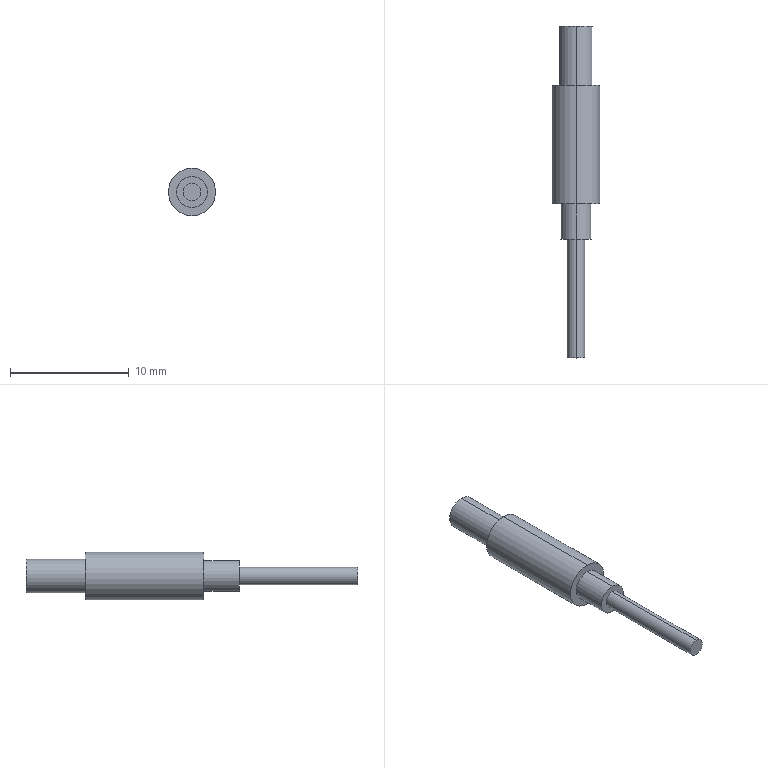Component | SolidWorks | FiberOpticHeadM4x10-1 | 1 solid | 13 faces | box 4 x 28 x 4 mm | volume 189 mm3 | cylinder 8 | plane 5 | commonest cylinder face diameters 2.8 x2 4 x2 2.6 x2 1.47 x2
build123d program:
from build123d import *


with BuildPart() as part:
    # Sketch1 → Revolve1 (revolve)
    with BuildSketch(Plane.XY, mode=Mode.PRIVATE) as revolve1_sk:
        Polygon((0, 0), (0.735, 0), (0.735, 10), (1.3, 10), (1.3, 13), (2, 13), (2, 23), (1.4, 23), (1.4, 28), (0, 28), align=None)
    revolve(revolve1_sk.sketch.rotate(Axis((0, 0, 0), (0, -1, 0)), 90), axis=Axis((0, 0, 0), (0, -1, 0)))


solid = part.part

# Placed as in the assembly
solid = solid.moved(Location((20.665, -23.632, -215.315), (0, 0, 0)))
STEP:
#1=COLOUR_RGB('',0.7922,0.8196,0.9333);
#2=FILL_AREA_STYLE_COLOUR('',#1);
#3=FILL_AREA_STYLE('',(#2));
#4=SURFACE_STYLE_FILL_AREA(#3);
#5=SURFACE_SIDE_STYLE('',(#4));
#6=SURFACE_STYLE_USAGE(.BOTH.,#5);
#7=PRESENTATION_STYLE_ASSIGNMENT((#6));
#8=CARTESIAN_POINT('',(0.8136,-0.02487,-8.422));
#9=VERTEX_POINT('',#8);
#10=CARTESIAN_POINT('',(0.8136,-0.02487,-8.532));
#11=VERTEX_POINT('',#10);
#12=CARTESIAN_POINT('',(0.8136,-0.02487,-8.477));
#13=DIRECTION('',(0.,1.,0.));
#14=DIRECTION('',(0.,0.,1.));
#15=AXIS2_PLACEMENT_3D('',#12,#13,#14);
#16=CIRCLE('',#15,0.05512);
#17=EDGE_CURVE('',#9,#11,#16,.T.);
#18=ORIENTED_EDGE('',*,*,#17,.T.);
#19=CARTESIAN_POINT('',(0.8136,0.172,-8.532));
#20=VERTEX_POINT('',#19);
#21=CARTESIAN_POINT('',(0.8136,-0.9304,-8.532));
#22=DIRECTION('',(0.,1.,0.));
#23=VECTOR('',#22,39.37);
#24=LINE('',#21,#23);
#25=EDGE_CURVE('',#11,#20,#24,.T.);
#26=ORIENTED_EDGE('',*,*,#25,.T.);
#27=CARTESIAN_POINT('',(0.8136,0.172,-8.422));
#28=VERTEX_POINT('',#27);
#29=CARTESIAN_POINT('',(0.8136,0.172,-8.477));
#30=DIRECTION('',(0.,1.,0.));
#31=DIRECTION('',(0.,0.,1.));
#32=AXIS2_PLACEMENT_3D('',#29,#30,#31);
#33=CIRCLE('',#32,0.05512);
#34=EDGE_CURVE('',#28,#20,#33,.T.);
#35=ORIENTED_EDGE('',*,*,#34,.F.);
#36=CARTESIAN_POINT('',(0.8136,-0.9304,-8.422));
#37=DIRECTION('',(0.,1.,0.));
#38=VECTOR('',#37,39.37);
#39=LINE('',#36,#38);
#40=EDGE_CURVE('',#9,#28,#39,.T.);
#41=ORIENTED_EDGE('',*,*,#40,.F.);
#42=EDGE_LOOP('',(#18,#26,#35,#41));
#43=FACE_OUTER_BOUND('',#42,.T.);
#44=CARTESIAN_POINT('',(0.8136,-0.9304,-8.477));
#45=DIRECTION('',(0.,1.,0.));
#46=DIRECTION('',(0.,0.,1.));
#47=AXIS2_PLACEMENT_3D('',#44,#45,#46);
#48=CYLINDRICAL_SURFACE('',#47,0.05512);
#49=ADVANCED_FACE('',(#43),#48,.T.);
#50=CARTESIAN_POINT('',(0.8136,-0.4186,-8.398));
#51=VERTEX_POINT('',#50);
#52=CARTESIAN_POINT('',(0.8136,-0.4186,-8.556));
#53=VERTEX_POINT('',#52);
#54=CARTESIAN_POINT('',(0.8136,-0.4186,-8.477));
#55=DIRECTION('',(0.,1.,0.));
#56=DIRECTION('',(0.,0.,1.));
#57=AXIS2_PLACEMENT_3D('',#54,#55,#56);
#58=CIRCLE('',#57,0.07874);
#59=EDGE_CURVE('',#51,#53,#58,.T.);
#60=ORIENTED_EDGE('',*,*,#59,.T.);
#61=CARTESIAN_POINT('',(0.8136,-0.02487,-8.556));
#62=VERTEX_POINT('',#61);
#63=CARTESIAN_POINT('',(0.8136,-0.9304,-8.556));
#64=DIRECTION('',(0.,1.,0.));
#65=VECTOR('',#64,39.37);
#66=LINE('',#63,#65);
#67=EDGE_CURVE('',#53,#62,#66,.T.);
#68=ORIENTED_EDGE('',*,*,#67,.T.);
#69=CARTESIAN_POINT('',(0.8136,-0.02487,-8.398));
#70=VERTEX_POINT('',#69);
#71=CARTESIAN_POINT('',(0.8136,-0.02487,-8.477));
#72=DIRECTION('',(0.,1.,0.));
#73=DIRECTION('',(0.,0.,1.));
#74=AXIS2_PLACEMENT_3D('',#71,#72,#73);
#75=CIRCLE('',#74,0.07874);
#76=EDGE_CURVE('',#70,#62,#75,.T.);
#77=ORIENTED_EDGE('',*,*,#76,.F.);
#78=CARTESIAN_POINT('',(0.8136,-0.9304,-8.398));
#79=DIRECTION('',(0.,1.,0.));
#80=VECTOR('',#79,39.37);
#81=LINE('',#78,#80);
#82=EDGE_CURVE('',#51,#70,#81,.T.);
#83=ORIENTED_EDGE('',*,*,#82,.F.);
#84=EDGE_LOOP('',(#60,#68,#77,#83));
#85=FACE_OUTER_BOUND('',#84,.T.);
#86=CARTESIAN_POINT('',(0.8136,-0.9304,-8.477));
#87=DIRECTION('',(0.,1.,0.));
#88=DIRECTION('',(0.,0.,1.));
#89=AXIS2_PLACEMENT_3D('',#86,#87,#88);
#90=CYLINDRICAL_SURFACE('',#89,0.07874);
#91=ADVANCED_FACE('',(#85),#90,.T.);
#92=CARTESIAN_POINT('',(0.8136,-0.5367,-8.426));
#93=VERTEX_POINT('',#92);
#94=CARTESIAN_POINT('',(0.8136,-0.5367,-8.528));
#95=VERTEX_POINT('',#94);
#96=CARTESIAN_POINT('',(0.8136,-0.5367,-8.477));
#97=DIRECTION('',(0.,1.,0.));
#98=DIRECTION('',(0.,0.,1.));
#99=AXIS2_PLACEMENT_3D('',#96,#97,#98);
#100=CIRCLE('',#99,0.05118);
#101=EDGE_CURVE('',#93,#95,#100,.T.);
#102=ORIENTED_EDGE('',*,*,#101,.T.);
#103=CARTESIAN_POINT('',(0.8136,-0.4186,-8.528));
#104=VERTEX_POINT('',#103);
#105=CARTESIAN_POINT('',(0.8136,-0.9304,-8.528));
#106=DIRECTION('',(0.,1.,0.));
#107=VECTOR('',#106,39.37);
#108=LINE('',#105,#107);
#109=EDGE_CURVE('',#95,#104,#108,.T.);
#110=ORIENTED_EDGE('',*,*,#109,.T.);
#111=CARTESIAN_POINT('',(0.8136,-0.4186,-8.426));
#112=VERTEX_POINT('',#111);
#113=CARTESIAN_POINT('',(0.8136,-0.4186,-8.477));
#114=DIRECTION('',(0.,1.,0.));
#115=DIRECTION('',(0.,0.,1.));
#116=AXIS2_PLACEMENT_3D('',#113,#114,#115);
#117=CIRCLE('',#116,0.05118);
#118=EDGE_CURVE('',#112,#104,#117,.T.);
#119=ORIENTED_EDGE('',*,*,#118,.F.);
#120=CARTESIAN_POINT('',(0.8136,-0.9304,-8.426));
#121=DIRECTION('',(0.,1.,0.));
#122=VECTOR('',#121,39.37);
#123=LINE('',#120,#122);
#124=EDGE_CURVE('',#93,#112,#123,.T.);
#125=ORIENTED_EDGE('',*,*,#124,.F.);
#126=EDGE_LOOP('',(#102,#110,#119,#125));
#127=FACE_OUTER_BOUND('',#126,.T.);
#128=CARTESIAN_POINT('',(0.8136,-0.9304,-8.477));
#129=DIRECTION('',(0.,1.,0.));
#130=DIRECTION('',(0.,0.,1.));
#131=AXIS2_PLACEMENT_3D('',#128,#129,#130);
#132=CYLINDRICAL_SURFACE('',#131,0.05118);
#133=ADVANCED_FACE('',(#127),#132,.T.);
#134=CARTESIAN_POINT('',(0.8136,-0.9304,-8.448));
#135=VERTEX_POINT('',#134);
#136=CARTESIAN_POINT('',(0.8136,-0.9304,-8.506));
#137=VERTEX_POINT('',#136);
#138=CARTESIAN_POINT('',(0.8136,-0.9304,-8.477));
#139=DIRECTION('',(0.,1.,0.));
#140=DIRECTION('',(0.,0.,1.));
#141=AXIS2_PLACEMENT_3D('',#138,#139,#140);
#142=CIRCLE('',#141,0.02894);
#143=EDGE_CURVE('',#135,#137,#142,.T.);
#144=ORIENTED_EDGE('',*,*,#143,.T.);
#145=CARTESIAN_POINT('',(0.8136,-0.5367,-8.506));
#146=VERTEX_POINT('',#145);
#147=CARTESIAN_POINT('',(0.8136,-0.9304,-8.506));
#148=DIRECTION('',(0.,1.,0.));
#149=VECTOR('',#148,39.37);
#150=LINE('',#147,#149);
#151=EDGE_CURVE('',#137,#146,#150,.T.);
#152=ORIENTED_EDGE('',*,*,#151,.T.);
#153=CARTESIAN_POINT('',(0.8136,-0.5367,-8.448));
#154=VERTEX_POINT('',#153);
#155=CARTESIAN_POINT('',(0.8136,-0.5367,-8.477));
#156=DIRECTION('',(0.,1.,0.));
#157=DIRECTION('',(0.,0.,1.));
#158=AXIS2_PLACEMENT_3D('',#155,#156,#157);
#159=CIRCLE('',#158,0.02894);
#160=EDGE_CURVE('',#154,#146,#159,.T.);
#161=ORIENTED_EDGE('',*,*,#160,.F.);
#162=CARTESIAN_POINT('',(0.8136,-0.9304,-8.448));
#163=DIRECTION('',(0.,1.,0.));
#164=VECTOR('',#163,39.37);
#165=LINE('',#162,#164);
#166=EDGE_CURVE('',#135,#154,#165,.T.);
#167=ORIENTED_EDGE('',*,*,#166,.F.);
#168=EDGE_LOOP('',(#144,#152,#161,#167));
#169=FACE_OUTER_BOUND('',#168,.T.);
#170=CARTESIAN_POINT('',(0.8136,-0.9304,-8.477));
#171=DIRECTION('',(0.,1.,0.));
#172=DIRECTION('',(0.,0.,1.));
#173=AXIS2_PLACEMENT_3D('',#170,#171,#172);
#174=CYLINDRICAL_SURFACE('',#173,0.02894);
#175=ADVANCED_FACE('',(#169),#174,.T.);
#176=ORIENTED_EDGE('',*,*,#143,.F.);
#177=CARTESIAN_POINT('',(0.8136,-0.9304,-8.477));
#178=DIRECTION('',(0.,1.,0.));
#179=DIRECTION('',(0.,0.,1.));
#180=AXIS2_PLACEMENT_3D('',#177,#178,#179);
#181=CIRCLE('',#180,0.02894);
#182=EDGE_CURVE('',#137,#135,#181,.T.);
#183=ORIENTED_EDGE('',*,*,#182,.F.);
#184=EDGE_LOOP('',(#176,#183));
#185=FACE_OUTER_BOUND('',#184,.T.);
#186=CARTESIAN_POINT('',(0.8136,-0.9304,-8.477));
#187=DIRECTION('',(0.,1.,0.));
#188=DIRECTION('',(0.,0.,1.));
#189=AXIS2_PLACEMENT_3D('',#186,#187,#188);
#190=PLANE('',#189);
#191=ADVANCED_FACE('',(#185),#190,.F.);
#192=ORIENTED_EDGE('',*,*,#151,.F.);
#193=ORIENTED_EDGE('',*,*,#182,.T.);
#194=ORIENTED_EDGE('',*,*,#166,.T.);
#195=CARTESIAN_POINT('',(0.8136,-0.5367,-8.477));
#196=DIRECTION('',(0.,1.,0.));
#197=DIRECTION('',(0.,0.,1.));
#198=AXIS2_PLACEMENT_3D('',#195,#196,#197);
#199=CIRCLE('',#198,0.02894);
#200=EDGE_CURVE('',#146,#154,#199,.T.);
#201=ORIENTED_EDGE('',*,*,#200,.F.);
#202=EDGE_LOOP('',(#192,#193,#194,#201));
#203=FACE_OUTER_BOUND('',#202,.T.);
#204=CARTESIAN_POINT('',(0.8136,-0.9304,-8.477));
#205=DIRECTION('',(0.,1.,0.));
#206=DIRECTION('',(0.,0.,1.));
#207=AXIS2_PLACEMENT_3D('',#204,#205,#206);
#208=CYLINDRICAL_SURFACE('',#207,0.02894);
#209=ADVANCED_FACE('',(#203),#208,.T.);
#210=ORIENTED_EDGE('',*,*,#101,.F.);
#211=CARTESIAN_POINT('',(0.8136,-0.5367,-8.477));
#212=DIRECTION('',(0.,1.,0.));
#213=DIRECTION('',(0.,0.,1.));
#214=AXIS2_PLACEMENT_3D('',#211,#212,#213);
#215=CIRCLE('',#214,0.05118);
#216=EDGE_CURVE('',#95,#93,#215,.T.);
#217=ORIENTED_EDGE('',*,*,#216,.F.);
#218=EDGE_LOOP('',(#210,#217));
#219=FACE_OUTER_BOUND('',#218,.T.);
#220=ORIENTED_EDGE('',*,*,#160,.T.);
#221=ORIENTED_EDGE('',*,*,#200,.T.);
#222=EDGE_LOOP('',(#220,#221));
#223=FACE_BOUND('',#222,.T.);
#224=CARTESIAN_POINT('',(0.8425,-0.5367,-8.477));
#225=DIRECTION('',(0.,1.,0.));
#226=DIRECTION('',(0.,0.,1.));
#227=AXIS2_PLACEMENT_3D('',#224,#225,#226);
#228=PLANE('',#227);
#229=ADVANCED_FACE('',(#219,#223),#228,.F.);
#230=ORIENTED_EDGE('',*,*,#109,.F.);
#231=ORIENTED_EDGE('',*,*,#216,.T.);
#232=ORIENTED_EDGE('',*,*,#124,.T.);
#233=CARTESIAN_POINT('',(0.8136,-0.4186,-8.477));
#234=DIRECTION('',(0.,1.,0.));
#235=DIRECTION('',(0.,0.,1.));
#236=AXIS2_PLACEMENT_3D('',#233,#234,#235);
#237=CIRCLE('',#236,0.05118);
#238=EDGE_CURVE('',#104,#112,#237,.T.);
#239=ORIENTED_EDGE('',*,*,#238,.F.);
#240=EDGE_LOOP('',(#230,#231,#232,#239));
#241=FACE_OUTER_BOUND('',#240,.T.);
#242=CARTESIAN_POINT('',(0.8136,-0.9304,-8.477));
#243=DIRECTION('',(0.,1.,0.));
#244=DIRECTION('',(0.,0.,1.));
#245=AXIS2_PLACEMENT_3D('',#242,#243,#244);
#246=CYLINDRICAL_SURFACE('',#245,0.05118);
#247=ADVANCED_FACE('',(#241),#246,.T.);
#248=ORIENTED_EDGE('',*,*,#59,.F.);
#249=CARTESIAN_POINT('',(0.8136,-0.4186,-8.477));
#250=DIRECTION('',(0.,1.,0.));
#251=DIRECTION('',(0.,0.,1.));
#252=AXIS2_PLACEMENT_3D('',#249,#250,#251);
#253=CIRCLE('',#252,0.07874);
#254=EDGE_CURVE('',#53,#51,#253,.T.);
#255=ORIENTED_EDGE('',*,*,#254,.F.);
#256=EDGE_LOOP('',(#248,#255));
#257=FACE_OUTER_BOUND('',#256,.T.);
#258=ORIENTED_EDGE('',*,*,#118,.T.);
#259=ORIENTED_EDGE('',*,*,#238,.T.);
#260=EDGE_LOOP('',(#258,#259));
#261=FACE_BOUND('',#260,.T.);
#262=CARTESIAN_POINT('',(0.8648,-0.4186,-8.477));
#263=DIRECTION('',(0.,1.,0.));
#264=DIRECTION('',(0.,0.,1.));
#265=AXIS2_PLACEMENT_3D('',#262,#263,#264);
#266=PLANE('',#265);
#267=ADVANCED_FACE('',(#257,#261),#266,.F.);
#268=ORIENTED_EDGE('',*,*,#67,.F.);
#269=ORIENTED_EDGE('',*,*,#254,.T.);
#270=ORIENTED_EDGE('',*,*,#82,.T.);
#271=CARTESIAN_POINT('',(0.8136,-0.02487,-8.477));
#272=DIRECTION('',(0.,1.,0.));
#273=DIRECTION('',(0.,0.,1.));
#274=AXIS2_PLACEMENT_3D('',#271,#272,#273);
#275=CIRCLE('',#274,0.07874);
#276=EDGE_CURVE('',#62,#70,#275,.T.);
#277=ORIENTED_EDGE('',*,*,#276,.F.);
#278=EDGE_LOOP('',(#268,#269,#270,#277));
#279=FACE_OUTER_BOUND('',#278,.T.);
#280=CARTESIAN_POINT('',(0.8136,-0.9304,-8.477));
#281=DIRECTION('',(0.,1.,0.));
#282=DIRECTION('',(0.,0.,1.));
#283=AXIS2_PLACEMENT_3D('',#280,#281,#282);
#284=CYLINDRICAL_SURFACE('',#283,0.07874);
#285=ADVANCED_FACE('',(#279),#284,.T.);
#286=ORIENTED_EDGE('',*,*,#17,.F.);
#287=CARTESIAN_POINT('',(0.8136,-0.02487,-8.477));
#288=DIRECTION('',(0.,1.,0.));
#289=DIRECTION('',(0.,0.,1.));
#290=AXIS2_PLACEMENT_3D('',#287,#288,#289);
#291=CIRCLE('',#290,0.05512);
#292=EDGE_CURVE('',#11,#9,#291,.T.);
#293=ORIENTED_EDGE('',*,*,#292,.F.);
#294=EDGE_LOOP('',(#286,#293));
#295=FACE_BOUND('',#294,.T.);
#296=ORIENTED_EDGE('',*,*,#76,.T.);
#297=ORIENTED_EDGE('',*,*,#276,.T.);
#298=EDGE_LOOP('',(#296,#297));
#299=FACE_OUTER_BOUND('',#298,.T.);
#300=CARTESIAN_POINT('',(0.8923,-0.02487,-8.477));
#301=DIRECTION('',(0.,-1.,0.));
#302=DIRECTION('',(0.,0.,-1.));
#303=AXIS2_PLACEMENT_3D('',#300,#301,#302);
#304=PLANE('',#303);
#305=ADVANCED_FACE('',(#295,#299),#304,.F.);
#306=ORIENTED_EDGE('',*,*,#25,.F.);
#307=ORIENTED_EDGE('',*,*,#292,.T.);
#308=ORIENTED_EDGE('',*,*,#40,.T.);
#309=CARTESIAN_POINT('',(0.8136,0.172,-8.477));
#310=DIRECTION('',(0.,1.,0.));
#311=DIRECTION('',(0.,0.,1.));
#312=AXIS2_PLACEMENT_3D('',#309,#310,#311);
#313=CIRCLE('',#312,0.05512);
#314=EDGE_CURVE('',#20,#28,#313,.T.);
#315=ORIENTED_EDGE('',*,*,#314,.F.);
#316=EDGE_LOOP('',(#306,#307,#308,#315));
#317=FACE_OUTER_BOUND('',#316,.T.);
#318=CARTESIAN_POINT('',(0.8136,-0.9304,-8.477));
#319=DIRECTION('',(0.,1.,0.));
#320=DIRECTION('',(0.,0.,1.));
#321=AXIS2_PLACEMENT_3D('',#318,#319,#320);
#322=CYLINDRICAL_SURFACE('',#321,0.05512);
#323=ADVANCED_FACE('',(#317),#322,.T.);
#324=ORIENTED_EDGE('',*,*,#34,.T.);
#325=ORIENTED_EDGE('',*,*,#314,.T.);
#326=EDGE_LOOP('',(#324,#325));
#327=FACE_OUTER_BOUND('',#326,.T.);
#328=CARTESIAN_POINT('',(0.8687,0.172,-8.477));
#329=DIRECTION('',(0.,-1.,0.));
#330=DIRECTION('',(0.,0.,-1.));
#331=AXIS2_PLACEMENT_3D('',#328,#329,#330);
#332=PLANE('',#331);
#333=ADVANCED_FACE('',(#327),#332,.F.);
#334=CLOSED_SHELL('',(#49,#91,#133,#175,#191,#209,#229,#247,#267,#285,#305,#323,#333));
#335=MANIFOLD_SOLID_BREP('',#334);
#336=STYLED_ITEM('',(#7),#335);
#337=(LENGTH_UNIT()NAMED_UNIT(*)SI_UNIT($,.METRE.));
#338=LENGTH_MEASURE_WITH_UNIT(LENGTH_MEASURE(0.0254),#337);
#339=DIMENSIONAL_EXPONENTS(1.,0.,0.,0.,0.,0.,0.);
#340=(CONVERSION_BASED_UNIT('',#338)LENGTH_UNIT()NAMED_UNIT(#339));
#341=UNCERTAINTY_MEASURE_WITH_UNIT(LENGTH_MEASURE(0.00001),#340,'','');
#342=(NAMED_UNIT(*)PLANE_ANGLE_UNIT()SI_UNIT($,.RADIAN.));
#343=(NAMED_UNIT(*)SI_UNIT($,.STERADIAN.)SOLID_ANGLE_UNIT());
#344=(GEOMETRIC_REPRESENTATION_CONTEXT(3)GLOBAL_UNCERTAINTY_ASSIGNED_CONTEXT((#341))GLOBAL_UNIT_ASSIGNED_CONTEXT((#340,#342,#343))REPRESENTATION_CONTEXT('',''));
#345=MECHANICAL_DESIGN_GEOMETRIC_PRESENTATION_REPRESENTATION('',(#336),#344);
#346=CARTESIAN_POINT('',(0.,0.,0.));
#347=DIRECTION('',(0.,0.,1.));
#348=DIRECTION('',(1.,0.,0.));
#349=AXIS2_PLACEMENT_3D('',#346,#347,#348);
#350=(LENGTH_UNIT()NAMED_UNIT(*)SI_UNIT($,.METRE.));
#351=LENGTH_MEASURE_WITH_UNIT(LENGTH_MEASURE(0.0254),#350);
#352=DIMENSIONAL_EXPONENTS(1.,0.,0.,0.,0.,0.,0.);
#353=(CONVERSION_BASED_UNIT('',#351)LENGTH_UNIT()NAMED_UNIT(#352));
#354=UNCERTAINTY_MEASURE_WITH_UNIT(LENGTH_MEASURE(0.00001),#353,'','');
#355=(NAMED_UNIT(*)PLANE_ANGLE_UNIT()SI_UNIT($,.RADIAN.));
#356=(NAMED_UNIT(*)SI_UNIT($,.STERADIAN.)SOLID_ANGLE_UNIT());
#357=(GEOMETRIC_REPRESENTATION_CONTEXT(3)GLOBAL_UNCERTAINTY_ASSIGNED_CONTEXT((#354))GLOBAL_UNIT_ASSIGNED_CONTEXT((#353,#355,#356))REPRESENTATION_CONTEXT('',''));
#358=ADVANCED_BREP_SHAPE_REPRESENTATION('',(#335,#349),#357);
#359=PRESENTATION_LAYER_ASSIGNMENT('','',(#336));